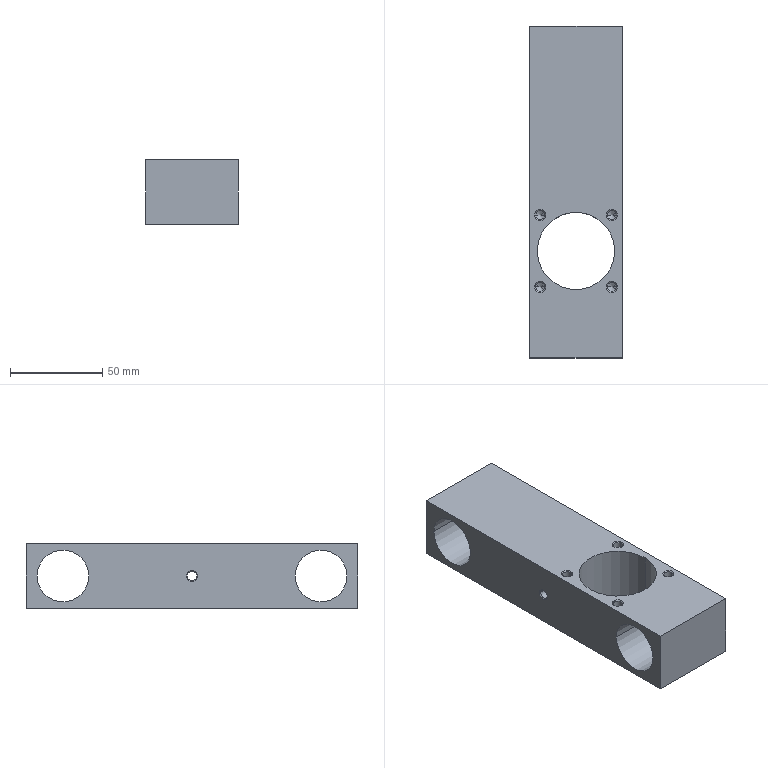Component | SolidWorks | DoubleFilmTransport-1_GuidePlate-1 | 1 solid | 40 faces | box 50 x 180 x 35 mm | volume 202252 mm3 | cone 18 | cylinder 16 | plane 6 | commonest cylinder face diameters 5 x10 28 x4 42 x2
STEP:
#1=COLOUR_RGB('',0.7922,0.8196,0.9333);
#2=FILL_AREA_STYLE_COLOUR('',#1);
#3=FILL_AREA_STYLE('',(#2));
#4=SURFACE_STYLE_FILL_AREA(#3);
#5=SURFACE_SIDE_STYLE('',(#4));
#6=SURFACE_STYLE_USAGE(.BOTH.,#5);
#7=PRESENTATION_STYLE_ASSIGNMENT((#6));
#8=CARTESIAN_POINT('',(-14.281,2.517,1.2));
#9=VERTEX_POINT('',#8);
#10=CARTESIAN_POINT('',(-14.478,2.517,1.2));
#11=VERTEX_POINT('',#10);
#12=CARTESIAN_POINT('',(-14.379,2.517,1.2));
#13=DIRECTION('',(0.,0.,1.));
#14=DIRECTION('',(-1.,0.,0.));
#15=AXIS2_PLACEMENT_3D('',#12,#13,#14);
#16=CIRCLE('',#15,0.09843);
#17=EDGE_CURVE('',#9,#11,#16,.T.);
#18=ORIENTED_EDGE('',*,*,#17,.F.);
#19=CARTESIAN_POINT('',(-14.26,2.517,1.22));
#20=VERTEX_POINT('',#19);
#21=CARTESIAN_POINT('',(-14.281,2.517,1.2));
#22=DIRECTION('',(0.7071,0.,0.7071));
#23=VECTOR('',#22,39.37);
#24=LINE('',#21,#23);
#25=EDGE_CURVE('',#9,#20,#24,.T.);
#26=ORIENTED_EDGE('',*,*,#25,.T.);
#27=CARTESIAN_POINT('',(-14.498,2.517,1.22));
#28=VERTEX_POINT('',#27);
#29=CARTESIAN_POINT('',(-14.379,2.517,1.22));
#30=DIRECTION('',(0.,0.,-1.));
#31=DIRECTION('',(-1.,0.,0.));
#32=AXIS2_PLACEMENT_3D('',#29,#30,#31);
#33=CIRCLE('',#32,0.1191);
#34=EDGE_CURVE('',#28,#20,#33,.T.);
#35=ORIENTED_EDGE('',*,*,#34,.F.);
#36=CARTESIAN_POINT('',(-14.478,2.517,1.2));
#37=DIRECTION('',(-0.7071,-0.,0.7071));
#38=VECTOR('',#37,39.37);
#39=LINE('',#36,#38);
#40=EDGE_CURVE('',#11,#28,#39,.T.);
#41=ORIENTED_EDGE('',*,*,#40,.F.);
#42=EDGE_LOOP('',(#18,#26,#35,#41));
#43=FACE_OUTER_BOUND('',#42,.T.);
#44=CARTESIAN_POINT('',(-14.379,2.517,1.2));
#45=DIRECTION('',(0.,0.,1.));
#46=DIRECTION('',(-1.,0.,0.));
#47=AXIS2_PLACEMENT_3D('',#44,#45,#46);
#48=CONICAL_SURFACE('',#47,0.09843,0.7854);
#49=ADVANCED_FACE('',(#43),#48,.F.);
#50=CARTESIAN_POINT('',(-15.812,2.517,1.2));
#51=VERTEX_POINT('',#50);
#52=CARTESIAN_POINT('',(-16.009,2.517,1.2));
#53=VERTEX_POINT('',#52);
#54=CARTESIAN_POINT('',(-15.91,2.517,1.2));
#55=DIRECTION('',(0.,0.,1.));
#56=DIRECTION('',(-1.,0.,0.));
#57=AXIS2_PLACEMENT_3D('',#54,#55,#56);
#58=CIRCLE('',#57,0.09843);
#59=EDGE_CURVE('',#51,#53,#58,.T.);
#60=ORIENTED_EDGE('',*,*,#59,.F.);
#61=CARTESIAN_POINT('',(-15.791,2.517,1.22));
#62=VERTEX_POINT('',#61);
#63=CARTESIAN_POINT('',(-15.812,2.517,1.2));
#64=DIRECTION('',(0.7071,0.,0.7071));
#65=VECTOR('',#64,39.37);
#66=LINE('',#63,#65);
#67=EDGE_CURVE('',#51,#62,#66,.T.);
#68=ORIENTED_EDGE('',*,*,#67,.T.);
#69=CARTESIAN_POINT('',(-16.029,2.517,1.22));
#70=VERTEX_POINT('',#69);
#71=CARTESIAN_POINT('',(-15.91,2.517,1.22));
#72=DIRECTION('',(0.,0.,-1.));
#73=DIRECTION('',(-1.,0.,0.));
#74=AXIS2_PLACEMENT_3D('',#71,#72,#73);
#75=CIRCLE('',#74,0.1191);
#76=EDGE_CURVE('',#70,#62,#75,.T.);
#77=ORIENTED_EDGE('',*,*,#76,.F.);
#78=CARTESIAN_POINT('',(-16.009,2.517,1.2));
#79=DIRECTION('',(-0.7071,-0.,0.7071));
#80=VECTOR('',#79,39.37);
#81=LINE('',#78,#80);
#82=EDGE_CURVE('',#53,#70,#81,.T.);
#83=ORIENTED_EDGE('',*,*,#82,.F.);
#84=EDGE_LOOP('',(#60,#68,#77,#83));
#85=FACE_OUTER_BOUND('',#84,.T.);
#86=CARTESIAN_POINT('',(-15.91,2.517,1.2));
#87=DIRECTION('',(0.,0.,1.));
#88=DIRECTION('',(-1.,0.,0.));
#89=AXIS2_PLACEMENT_3D('',#86,#87,#88);
#90=CONICAL_SURFACE('',#89,0.09843,0.7854);
#91=ADVANCED_FACE('',(#85),#90,.F.);
#92=CARTESIAN_POINT('',(-16.108,4.641,0.5315));
#93=VERTEX_POINT('',#92);
#94=CARTESIAN_POINT('',(-16.108,4.444,0.5315));
#95=VERTEX_POINT('',#94);
#96=CARTESIAN_POINT('',(-16.108,4.542,0.5315));
#97=DIRECTION('',(-1.,-0.,0.));
#98=DIRECTION('',(0.,-1.,0.));
#99=AXIS2_PLACEMENT_3D('',#96,#97,#98);
#100=CIRCLE('',#99,0.09843);
#101=EDGE_CURVE('',#93,#95,#100,.T.);
#102=ORIENTED_EDGE('',*,*,#101,.F.);
#103=CARTESIAN_POINT('',(-16.129,4.661,0.5315));
#104=VERTEX_POINT('',#103);
#105=CARTESIAN_POINT('',(-16.108,4.641,0.5315));
#106=DIRECTION('',(-0.7071,0.7071,0.));
#107=VECTOR('',#106,39.37);
#108=LINE('',#105,#107);
#109=EDGE_CURVE('',#93,#104,#108,.T.);
#110=ORIENTED_EDGE('',*,*,#109,.T.);
#111=CARTESIAN_POINT('',(-16.129,4.423,0.5315));
#112=VERTEX_POINT('',#111);
#113=CARTESIAN_POINT('',(-16.129,4.542,0.5315));
#114=DIRECTION('',(1.,0.,0.));
#115=DIRECTION('',(0.,-1.,0.));
#116=AXIS2_PLACEMENT_3D('',#113,#114,#115);
#117=CIRCLE('',#116,0.1191);
#118=EDGE_CURVE('',#112,#104,#117,.T.);
#119=ORIENTED_EDGE('',*,*,#118,.F.);
#120=CARTESIAN_POINT('',(-16.108,4.444,0.5315));
#121=DIRECTION('',(-0.7071,-0.7071,0.));
#122=VECTOR('',#121,39.37);
#123=LINE('',#120,#122);
#124=EDGE_CURVE('',#95,#112,#123,.T.);
#125=ORIENTED_EDGE('',*,*,#124,.F.);
#126=EDGE_LOOP('',(#102,#110,#119,#125));
#127=FACE_OUTER_BOUND('',#126,.T.);
#128=CARTESIAN_POINT('',(-16.108,4.542,0.5315));
#129=DIRECTION('',(-1.,-0.,0.));
#130=DIRECTION('',(0.,-1.,0.));
#131=AXIS2_PLACEMENT_3D('',#128,#129,#130);
#132=CONICAL_SURFACE('',#131,0.09843,0.7854);
#133=ADVANCED_FACE('',(#127),#132,.F.);
#134=CARTESIAN_POINT('',(-15.812,4.048,1.2));
#135=VERTEX_POINT('',#134);
#136=CARTESIAN_POINT('',(-16.009,4.048,1.2));
#137=VERTEX_POINT('',#136);
#138=CARTESIAN_POINT('',(-15.91,4.048,1.2));
#139=DIRECTION('',(0.,0.,1.));
#140=DIRECTION('',(-1.,0.,0.));
#141=AXIS2_PLACEMENT_3D('',#138,#139,#140);
#142=CIRCLE('',#141,0.09843);
#143=EDGE_CURVE('',#135,#137,#142,.T.);
#144=ORIENTED_EDGE('',*,*,#143,.F.);
#145=CARTESIAN_POINT('',(-15.791,4.048,1.22));
#146=VERTEX_POINT('',#145);
#147=CARTESIAN_POINT('',(-15.812,4.048,1.2));
#148=DIRECTION('',(0.7071,0.,0.7071));
#149=VECTOR('',#148,39.37);
#150=LINE('',#147,#149);
#151=EDGE_CURVE('',#135,#146,#150,.T.);
#152=ORIENTED_EDGE('',*,*,#151,.T.);
#153=CARTESIAN_POINT('',(-16.029,4.048,1.22));
#154=VERTEX_POINT('',#153);
#155=CARTESIAN_POINT('',(-15.91,4.048,1.22));
#156=DIRECTION('',(0.,0.,-1.));
#157=DIRECTION('',(-1.,0.,0.));
#158=AXIS2_PLACEMENT_3D('',#155,#156,#157);
#159=CIRCLE('',#158,0.1191);
#160=EDGE_CURVE('',#154,#146,#159,.T.);
#161=ORIENTED_EDGE('',*,*,#160,.F.);
#162=CARTESIAN_POINT('',(-16.009,4.048,1.2));
#163=DIRECTION('',(-0.7071,-0.,0.7071));
#164=VECTOR('',#163,39.37);
#165=LINE('',#162,#164);
#166=EDGE_CURVE('',#137,#154,#165,.T.);
#167=ORIENTED_EDGE('',*,*,#166,.F.);
#168=EDGE_LOOP('',(#144,#152,#161,#167));
#169=FACE_OUTER_BOUND('',#168,.T.);
#170=CARTESIAN_POINT('',(-15.91,4.048,1.2));
#171=DIRECTION('',(0.,0.,1.));
#172=DIRECTION('',(-1.,0.,0.));
#173=AXIS2_PLACEMENT_3D('',#170,#171,#172);
#174=CONICAL_SURFACE('',#173,0.09843,0.7854);
#175=ADVANCED_FACE('',(#169),#174,.F.);
#176=CARTESIAN_POINT('',(-14.281,4.048,1.2));
#177=VERTEX_POINT('',#176);
#178=CARTESIAN_POINT('',(-14.478,4.048,1.2));
#179=VERTEX_POINT('',#178);
#180=CARTESIAN_POINT('',(-14.379,4.048,1.2));
#181=DIRECTION('',(0.,0.,1.));
#182=DIRECTION('',(-1.,0.,0.));
#183=AXIS2_PLACEMENT_3D('',#180,#181,#182);
#184=CIRCLE('',#183,0.09843);
#185=EDGE_CURVE('',#177,#179,#184,.T.);
#186=ORIENTED_EDGE('',*,*,#185,.F.);
#187=CARTESIAN_POINT('',(-14.26,4.048,1.22));
#188=VERTEX_POINT('',#187);
#189=CARTESIAN_POINT('',(-14.281,4.048,1.2));
#190=DIRECTION('',(0.7071,0.,0.7071));
#191=VECTOR('',#190,39.37);
#192=LINE('',#189,#191);
#193=EDGE_CURVE('',#177,#188,#192,.T.);
#194=ORIENTED_EDGE('',*,*,#193,.T.);
#195=CARTESIAN_POINT('',(-14.498,4.048,1.22));
#196=VERTEX_POINT('',#195);
#197=CARTESIAN_POINT('',(-14.379,4.048,1.22));
#198=DIRECTION('',(0.,0.,-1.));
#199=DIRECTION('',(-1.,0.,0.));
#200=AXIS2_PLACEMENT_3D('',#197,#198,#199);
#201=CIRCLE('',#200,0.1191);
#202=EDGE_CURVE('',#196,#188,#201,.T.);
#203=ORIENTED_EDGE('',*,*,#202,.F.);
#204=CARTESIAN_POINT('',(-14.478,4.048,1.2));
#205=DIRECTION('',(-0.7071,-0.,0.7071));
#206=VECTOR('',#205,39.37);
#207=LINE('',#204,#206);
#208=EDGE_CURVE('',#179,#196,#207,.T.);
#209=ORIENTED_EDGE('',*,*,#208,.F.);
#210=EDGE_LOOP('',(#186,#194,#203,#209));
#211=FACE_OUTER_BOUND('',#210,.T.);
#212=CARTESIAN_POINT('',(-14.379,4.048,1.2));
#213=DIRECTION('',(0.,0.,1.));
#214=DIRECTION('',(-1.,0.,0.));
#215=AXIS2_PLACEMENT_3D('',#212,#213,#214);
#216=CONICAL_SURFACE('',#215,0.09843,0.7854);
#217=ADVANCED_FACE('',(#211),#216,.F.);
#218=CARTESIAN_POINT('',(-15.812,4.048,0.3937));
#219=VERTEX_POINT('',#218);
#220=CARTESIAN_POINT('',(-16.009,4.048,0.3937));
#221=VERTEX_POINT('',#220);
#222=CARTESIAN_POINT('',(-15.91,4.048,0.3937));
#223=DIRECTION('',(0.,0.,1.));
#224=DIRECTION('',(-1.,0.,0.));
#225=AXIS2_PLACEMENT_3D('',#222,#223,#224);
#226=CIRCLE('',#225,0.09843);
#227=EDGE_CURVE('',#219,#221,#226,.T.);
#228=ORIENTED_EDGE('',*,*,#227,.F.);
#229=CARTESIAN_POINT('',(-15.812,4.048,1.22));
#230=DIRECTION('',(0.,0.,1.));
#231=VECTOR('',#230,39.37);
#232=LINE('',#229,#231);
#233=EDGE_CURVE('',#219,#135,#232,.T.);
#234=ORIENTED_EDGE('',*,*,#233,.T.);
#235=ORIENTED_EDGE('',*,*,#143,.T.);
#236=CARTESIAN_POINT('',(-16.009,4.048,1.22));
#237=DIRECTION('',(0.,0.,1.));
#238=VECTOR('',#237,39.37);
#239=LINE('',#236,#238);
#240=EDGE_CURVE('',#221,#137,#239,.T.);
#241=ORIENTED_EDGE('',*,*,#240,.F.);
#242=EDGE_LOOP('',(#228,#234,#235,#241));
#243=FACE_OUTER_BOUND('',#242,.T.);
#244=CARTESIAN_POINT('',(-15.91,4.048,1.22));
#245=DIRECTION('',(0.,0.,1.));
#246=DIRECTION('',(-1.,0.,0.));
#247=AXIS2_PLACEMENT_3D('',#244,#245,#246);
#248=CYLINDRICAL_SURFACE('',#247,0.09843);
#249=ADVANCED_FACE('',(#243),#248,.F.);
#250=CARTESIAN_POINT('',(-15.91,4.048,0.3346));
#251=VERTEX_POINT('',#250);
#252=CARTESIAN_POINT('',(-16.009,4.048,0.3937));
#253=DIRECTION('',(-0.8572,-0.,0.515));
#254=VECTOR('',#253,39.37);
#255=LINE('',#252,#254);
#256=EDGE_CURVE('',#251,#221,#255,.T.);
#257=ORIENTED_EDGE('',*,*,#256,.F.);
#258=CARTESIAN_POINT('',(-15.812,4.048,0.3937));
#259=DIRECTION('',(0.8572,0.,0.515));
#260=VECTOR('',#259,39.37);
#261=LINE('',#258,#260);
#262=EDGE_CURVE('',#251,#219,#261,.T.);
#263=ORIENTED_EDGE('',*,*,#262,.T.);
#264=ORIENTED_EDGE('',*,*,#227,.T.);
#265=EDGE_LOOP('',(#257,#263,#264));
#266=FACE_OUTER_BOUND('',#265,.T.);
#267=CARTESIAN_POINT('',(-15.91,4.048,0.3937));
#268=DIRECTION('',(0.,0.,1.));
#269=DIRECTION('',(-1.,0.,0.));
#270=AXIS2_PLACEMENT_3D('',#267,#268,#269);
#271=CONICAL_SURFACE('',#270,0.09843,1.03);
#272=ADVANCED_FACE('',(#266),#271,.F.);
#273=CARTESIAN_POINT('',(-15.812,2.517,0.3937));
#274=VERTEX_POINT('',#273);
#275=CARTESIAN_POINT('',(-16.009,2.517,0.3937));
#276=VERTEX_POINT('',#275);
#277=CARTESIAN_POINT('',(-15.91,2.517,0.3937));
#278=DIRECTION('',(0.,0.,1.));
#279=DIRECTION('',(-1.,0.,0.));
#280=AXIS2_PLACEMENT_3D('',#277,#278,#279);
#281=CIRCLE('',#280,0.09843);
#282=EDGE_CURVE('',#274,#276,#281,.T.);
#283=ORIENTED_EDGE('',*,*,#282,.F.);
#284=CARTESIAN_POINT('',(-15.812,2.517,1.22));
#285=DIRECTION('',(0.,0.,1.));
#286=VECTOR('',#285,39.37);
#287=LINE('',#284,#286);
#288=EDGE_CURVE('',#274,#51,#287,.T.);
#289=ORIENTED_EDGE('',*,*,#288,.T.);
#290=ORIENTED_EDGE('',*,*,#59,.T.);
#291=CARTESIAN_POINT('',(-16.009,2.517,1.22));
#292=DIRECTION('',(0.,0.,1.));
#293=VECTOR('',#292,39.37);
#294=LINE('',#291,#293);
#295=EDGE_CURVE('',#276,#53,#294,.T.);
#296=ORIENTED_EDGE('',*,*,#295,.F.);
#297=EDGE_LOOP('',(#283,#289,#290,#296));
#298=FACE_OUTER_BOUND('',#297,.T.);
#299=CARTESIAN_POINT('',(-15.91,2.517,1.22));
#300=DIRECTION('',(0.,0.,1.));
#301=DIRECTION('',(-1.,0.,0.));
#302=AXIS2_PLACEMENT_3D('',#299,#300,#301);
#303=CYLINDRICAL_SURFACE('',#302,0.09843);
#304=ADVANCED_FACE('',(#298),#303,.F.);
#305=CARTESIAN_POINT('',(-15.91,2.517,0.3346));
#306=VERTEX_POINT('',#305);
#307=CARTESIAN_POINT('',(-16.009,2.517,0.3937));
#308=DIRECTION('',(-0.8572,-0.,0.515));
#309=VECTOR('',#308,39.37);
#310=LINE('',#307,#309);
#311=EDGE_CURVE('',#306,#276,#310,.T.);
#312=ORIENTED_EDGE('',*,*,#311,.F.);
#313=CARTESIAN_POINT('',(-15.812,2.517,0.3937));
#314=DIRECTION('',(0.8572,0.,0.515));
#315=VECTOR('',#314,39.37);
#316=LINE('',#313,#315);
#317=EDGE_CURVE('',#306,#274,#316,.T.);
#318=ORIENTED_EDGE('',*,*,#317,.T.);
#319=ORIENTED_EDGE('',*,*,#282,.T.);
#320=EDGE_LOOP('',(#312,#318,#319));
#321=FACE_OUTER_BOUND('',#320,.T.);
#322=CARTESIAN_POINT('',(-15.91,2.517,0.3937));
#323=DIRECTION('',(0.,0.,1.));
#324=DIRECTION('',(-1.,0.,0.));
#325=AXIS2_PLACEMENT_3D('',#322,#323,#324);
#326=CONICAL_SURFACE('',#325,0.09843,1.03);
#327=ADVANCED_FACE('',(#321),#326,.F.);
#328=CARTESIAN_POINT('',(-14.281,2.517,0.3937));
#329=VERTEX_POINT('',#328);
#330=CARTESIAN_POINT('',(-14.478,2.517,0.3937));
#331=VERTEX_POINT('',#330);
#332=CARTESIAN_POINT('',(-14.379,2.517,0.3937));
#333=DIRECTION('',(0.,0.,1.));
#334=DIRECTION('',(-1.,0.,0.));
#335=AXIS2_PLACEMENT_3D('',#332,#333,#334);
#336=CIRCLE('',#335,0.09843);
#337=EDGE_CURVE('',#329,#331,#336,.T.);
#338=ORIENTED_EDGE('',*,*,#337,.F.);
#339=CARTESIAN_POINT('',(-14.281,2.517,1.22));
#340=DIRECTION('',(0.,0.,1.));
#341=VECTOR('',#340,39.37);
#342=LINE('',#339,#341);
#343=EDGE_CURVE('',#329,#9,#342,.T.);
#344=ORIENTED_EDGE('',*,*,#343,.T.);
#345=ORIENTED_EDGE('',*,*,#17,.T.);
#346=CARTESIAN_POINT('',(-14.478,2.517,1.22));
#347=DIRECTION('',(0.,0.,1.));
#348=VECTOR('',#347,39.37);
#349=LINE('',#346,#348);
#350=EDGE_CURVE('',#331,#11,#349,.T.);
#351=ORIENTED_EDGE('',*,*,#350,.F.);
#352=EDGE_LOOP('',(#338,#344,#345,#351));
#353=FACE_OUTER_BOUND('',#352,.T.);
#354=CARTESIAN_POINT('',(-14.379,2.517,1.22));
#355=DIRECTION('',(0.,0.,1.));
#356=DIRECTION('',(-1.,0.,0.));
#357=AXIS2_PLACEMENT_3D('',#354,#355,#356);
#358=CYLINDRICAL_SURFACE('',#357,0.09843);
#359=ADVANCED_FACE('',(#353),#358,.F.);
#360=CARTESIAN_POINT('',(-14.379,2.517,0.3346));
#361=VERTEX_POINT('',#360);
#362=CARTESIAN_POINT('',(-14.478,2.517,0.3937));
#363=DIRECTION('',(-0.8572,-0.,0.515));
#364=VECTOR('',#363,39.37);
#365=LINE('',#362,#364);
#366=EDGE_CURVE('',#361,#331,#365,.T.);
#367=ORIENTED_EDGE('',*,*,#366,.F.);
#368=CARTESIAN_POINT('',(-14.281,2.517,0.3937));
#369=DIRECTION('',(0.8572,0.,0.515));
#370=VECTOR('',#369,39.37);
#371=LINE('',#368,#370);
#372=EDGE_CURVE('',#361,#329,#371,.T.);
#373=ORIENTED_EDGE('',*,*,#372,.T.);
#374=ORIENTED_EDGE('',*,*,#337,.T.);
#375=EDGE_LOOP('',(#367,#373,#374));
#376=FACE_OUTER_BOUND('',#375,.T.);
#377=CARTESIAN_POINT('',(-14.379,2.517,0.3937));
#378=DIRECTION('',(0.,0.,1.));
#379=DIRECTION('',(-1.,0.,0.));
#380=AXIS2_PLACEMENT_3D('',#377,#378,#379);
#381=CONICAL_SURFACE('',#380,0.09843,1.03);
#382=ADVANCED_FACE('',(#376),#381,.F.);
#383=CARTESIAN_POINT('',(-14.281,4.048,0.3937));
#384=VERTEX_POINT('',#383);
#385=CARTESIAN_POINT('',(-14.478,4.048,0.3937));
#386=VERTEX_POINT('',#385);
#387=CARTESIAN_POINT('',(-14.379,4.048,0.3937));
#388=DIRECTION('',(0.,0.,1.));
#389=DIRECTION('',(-1.,0.,0.));
#390=AXIS2_PLACEMENT_3D('',#387,#388,#389);
#391=CIRCLE('',#390,0.09843);
#392=EDGE_CURVE('',#384,#386,#391,.T.);
#393=ORIENTED_EDGE('',*,*,#392,.F.);
#394=CARTESIAN_POINT('',(-14.281,4.048,1.22));
#395=DIRECTION('',(0.,0.,1.));
#396=VECTOR('',#395,39.37);
#397=LINE('',#394,#396);
#398=EDGE_CURVE('',#384,#177,#397,.T.);
#399=ORIENTED_EDGE('',*,*,#398,.T.);
#400=ORIENTED_EDGE('',*,*,#185,.T.);
#401=CARTESIAN_POINT('',(-14.478,4.048,1.22));
#402=DIRECTION('',(0.,0.,1.));
#403=VECTOR('',#402,39.37);
#404=LINE('',#401,#403);
#405=EDGE_CURVE('',#386,#179,#404,.T.);
#406=ORIENTED_EDGE('',*,*,#405,.F.);
#407=EDGE_LOOP('',(#393,#399,#400,#406));
#408=FACE_OUTER_BOUND('',#407,.T.);
#409=CARTESIAN_POINT('',(-14.379,4.048,1.22));
#410=DIRECTION('',(0.,0.,1.));
#411=DIRECTION('',(-1.,0.,0.));
#412=AXIS2_PLACEMENT_3D('',#409,#410,#411);
#413=CYLINDRICAL_SURFACE('',#412,0.09843);
#414=ADVANCED_FACE('',(#408),#413,.F.);
#415=CARTESIAN_POINT('',(-14.379,4.048,0.3346));
#416=VERTEX_POINT('',#415);
#417=CARTESIAN_POINT('',(-14.478,4.048,0.3937));
#418=DIRECTION('',(-0.8572,-0.,0.515));
#419=VECTOR('',#418,39.37);
#420=LINE('',#417,#419);
#421=EDGE_CURVE('',#416,#386,#420,.T.);
#422=ORIENTED_EDGE('',*,*,#421,.F.);
#423=CARTESIAN_POINT('',(-14.281,4.048,0.3937));
#424=DIRECTION('',(0.8572,0.,0.515));
#425=VECTOR('',#424,39.37);
#426=LINE('',#423,#425);
#427=EDGE_CURVE('',#416,#384,#426,.T.);
#428=ORIENTED_EDGE('',*,*,#427,.T.);
#429=ORIENTED_EDGE('',*,*,#392,.T.);
#430=EDGE_LOOP('',(#422,#428,#429));
#431=FACE_OUTER_BOUND('',#430,.T.);
#432=CARTESIAN_POINT('',(-14.379,4.048,0.3937));
#433=DIRECTION('',(0.,0.,1.));
#434=DIRECTION('',(-1.,0.,0.));
#435=AXIS2_PLACEMENT_3D('',#432,#433,#434);
#436=CONICAL_SURFACE('',#435,0.09843,1.03);
#437=ADVANCED_FACE('',(#431),#436,.F.);
#438=CARTESIAN_POINT('',(-14.161,4.641,0.5315));
#439=VERTEX_POINT('',#438);
#440=CARTESIAN_POINT('',(-14.161,4.444,0.5315));
#441=VERTEX_POINT('',#440);
#442=CARTESIAN_POINT('',(-14.161,4.542,0.5315));
#443=DIRECTION('',(-1.,-0.,0.));
#444=DIRECTION('',(0.,-1.,0.));
#445=AXIS2_PLACEMENT_3D('',#442,#443,#444);
#446=CIRCLE('',#445,0.09843);
#447=EDGE_CURVE('',#439,#441,#446,.T.);
#448=ORIENTED_EDGE('',*,*,#447,.F.);
#449=CARTESIAN_POINT('',(-16.129,4.641,0.5315));
#450=DIRECTION('',(-1.,-0.,0.));
#451=VECTOR('',#450,39.37);
#452=LINE('',#449,#451);
#453=EDGE_CURVE('',#439,#93,#452,.T.);
#454=ORIENTED_EDGE('',*,*,#453,.T.);
#455=ORIENTED_EDGE('',*,*,#101,.T.);
#456=CARTESIAN_POINT('',(-16.129,4.444,0.5315));
#457=DIRECTION('',(-1.,-0.,0.));
#458=VECTOR('',#457,39.37);
#459=LINE('',#456,#458);
#460=EDGE_CURVE('',#441,#95,#459,.T.);
#461=ORIENTED_EDGE('',*,*,#460,.F.);
#462=EDGE_LOOP('',(#448,#454,#455,#461));
#463=FACE_OUTER_BOUND('',#462,.T.);
#464=CARTESIAN_POINT('',(-16.129,4.542,0.5315));
#465=DIRECTION('',(-1.,-0.,0.));
#466=DIRECTION('',(0.,-1.,0.));
#467=AXIS2_PLACEMENT_3D('',#464,#465,#466);
#468=CYLINDRICAL_SURFACE('',#467,0.09843);
#469=ADVANCED_FACE('',(#463),#468,.F.);
#470=CARTESIAN_POINT('',(-14.161,2.338,0.5315));
#471=VERTEX_POINT('',#470);
#472=CARTESIAN_POINT('',(-14.161,1.235,0.5315));
#473=VERTEX_POINT('',#472);
#474=CARTESIAN_POINT('',(-14.161,1.786,0.5315));
#475=DIRECTION('',(-1.,-0.,0.));
#476=DIRECTION('',(0.,-1.,0.));
#477=AXIS2_PLACEMENT_3D('',#474,#475,#476);
#478=CIRCLE('',#477,0.5512);
#479=EDGE_CURVE('',#471,#473,#478,.T.);
#480=ORIENTED_EDGE('',*,*,#479,.F.);
#481=CARTESIAN_POINT('',(-16.129,2.338,0.5315));
#482=VERTEX_POINT('',#481);
#483=CARTESIAN_POINT('',(-16.129,2.338,0.5315));
#484=DIRECTION('',(-1.,-0.,0.));
#485=VECTOR('',#484,39.37);
#486=LINE('',#483,#485);
#487=EDGE_CURVE('',#471,#482,#486,.T.);
#488=ORIENTED_EDGE('',*,*,#487,.T.);
#489=CARTESIAN_POINT('',(-16.129,1.235,0.5315));
#490=VERTEX_POINT('',#489);
#491=CARTESIAN_POINT('',(-16.129,1.786,0.5315));
#492=DIRECTION('',(-1.,-0.,0.));
#493=DIRECTION('',(0.,-1.,0.));
#494=AXIS2_PLACEMENT_3D('',#491,#492,#493);
#495=CIRCLE('',#494,0.5512);
#496=EDGE_CURVE('',#482,#490,#495,.T.);
#497=ORIENTED_EDGE('',*,*,#496,.T.);
#498=CARTESIAN_POINT('',(-16.129,1.235,0.5315));
#499=DIRECTION('',(-1.,-0.,0.));
#500=VECTOR('',#499,39.37);
#501=LINE('',#498,#500);
#502=EDGE_CURVE('',#473,#490,#501,.T.);
#503=ORIENTED_EDGE('',*,*,#502,.F.);
#504=EDGE_LOOP('',(#480,#488,#497,#503));
#505=FACE_OUTER_BOUND('',#504,.T.);
#506=CARTESIAN_POINT('',(-16.129,1.786,0.5315));
#507=DIRECTION('',(-1.,-0.,0.));
#508=DIRECTION('',(0.,-1.,0.));
#509=AXIS2_PLACEMENT_3D('',#506,#507,#508);
#510=CYLINDRICAL_SURFACE('',#509,0.5512);
#511=ADVANCED_FACE('',(#505),#510,.F.);
#512=CARTESIAN_POINT('',(-14.161,7.849,0.5315));
#513=VERTEX_POINT('',#512);
#514=CARTESIAN_POINT('',(-14.161,6.747,0.5315));
#515=VERTEX_POINT('',#514);
#516=CARTESIAN_POINT('',(-14.161,7.298,0.5315));
#517=DIRECTION('',(-1.,-0.,0.));
#518=DIRECTION('',(0.,-1.,0.));
#519=AXIS2_PLACEMENT_3D('',#516,#517,#518);
#520=CIRCLE('',#519,0.5512);
#521=EDGE_CURVE('',#513,#515,#520,.T.);
#522=ORIENTED_EDGE('',*,*,#521,.F.);
#523=CARTESIAN_POINT('',(-16.129,7.849,0.5315));
#524=VERTEX_POINT('',#523);
#525=CARTESIAN_POINT('',(-16.129,7.849,0.5315));
#526=DIRECTION('',(-1.,-0.,0.));
#527=VECTOR('',#526,39.37);
#528=LINE('',#525,#527);
#529=EDGE_CURVE('',#513,#524,#528,.T.);
#530=ORIENTED_EDGE('',*,*,#529,.T.);
#531=CARTESIAN_POINT('',(-16.129,6.747,0.5315));
#532=VERTEX_POINT('',#531);
#533=CARTESIAN_POINT('',(-16.129,7.298,0.5315));
#534=DIRECTION('',(-1.,-0.,0.));
#535=DIRECTION('',(0.,-1.,0.));
#536=AXIS2_PLACEMENT_3D('',#533,#534,#535);
#537=CIRCLE('',#536,0.5512);
#538=EDGE_CURVE('',#524,#532,#537,.T.);
#539=ORIENTED_EDGE('',*,*,#538,.T.);
#540=CARTESIAN_POINT('',(-16.129,6.747,0.5315));
#541=DIRECTION('',(-1.,-0.,0.));
#542=VECTOR('',#541,39.37);
#543=LINE('',#540,#542);
#544=EDGE_CURVE('',#515,#532,#543,.T.);
#545=ORIENTED_EDGE('',*,*,#544,.F.);
#546=EDGE_LOOP('',(#522,#530,#539,#545));
#547=FACE_OUTER_BOUND('',#546,.T.);
#548=CARTESIAN_POINT('',(-16.129,7.298,0.5315));
#549=DIRECTION('',(-1.,-0.,0.));
#550=DIRECTION('',(0.,-1.,0.));
#551=AXIS2_PLACEMENT_3D('',#548,#549,#550);
#552=CYLINDRICAL_SURFACE('',#551,0.5512);
#553=ADVANCED_FACE('',(#547),#552,.F.);
#554=CARTESIAN_POINT('',(-15.972,3.282,1.22));
#555=VERTEX_POINT('',#554);
#556=CARTESIAN_POINT('',(-14.318,3.282,1.22));
#557=VERTEX_POINT('',#556);
#558=CARTESIAN_POINT('',(-15.145,3.282,1.22));
#559=DIRECTION('',(0.,0.,-1.));
#560=DIRECTION('',(1.,0.,0.));
#561=AXIS2_PLACEMENT_3D('',#558,#559,#560);
#562=CIRCLE('',#561,0.8268);
#563=EDGE_CURVE('',#555,#557,#562,.T.);
#564=ORIENTED_EDGE('',*,*,#563,.F.);
#565=CARTESIAN_POINT('',(-15.972,3.282,-0.1575));
#566=VERTEX_POINT('',#565);
#567=CARTESIAN_POINT('',(-15.972,3.282,-0.1575));
#568=DIRECTION('',(0.,0.,-1.));
#569=VECTOR('',#568,39.37);
#570=LINE('',#567,#569);
#571=EDGE_CURVE('',#555,#566,#570,.T.);
#572=ORIENTED_EDGE('',*,*,#571,.T.);
#573=CARTESIAN_POINT('',(-14.318,3.282,-0.1575));
#574=VERTEX_POINT('',#573);
#575=CARTESIAN_POINT('',(-15.145,3.282,-0.1575));
#576=DIRECTION('',(0.,0.,-1.));
#577=DIRECTION('',(1.,0.,0.));
#578=AXIS2_PLACEMENT_3D('',#575,#576,#577);
#579=CIRCLE('',#578,0.8268);
#580=EDGE_CURVE('',#566,#574,#579,.T.);
#581=ORIENTED_EDGE('',*,*,#580,.T.);
#582=CARTESIAN_POINT('',(-14.318,3.282,-0.1575));
#583=DIRECTION('',(0.,0.,-1.));
#584=VECTOR('',#583,39.37);
#585=LINE('',#582,#584);
#586=EDGE_CURVE('',#557,#574,#585,.T.);
#587=ORIENTED_EDGE('',*,*,#586,.F.);
#588=EDGE_LOOP('',(#564,#572,#581,#587));
#589=FACE_OUTER_BOUND('',#588,.T.);
#590=CARTESIAN_POINT('',(-15.145,3.282,-0.1575));
#591=DIRECTION('',(0.,0.,-1.));
#592=DIRECTION('',(1.,0.,0.));
#593=AXIS2_PLACEMENT_3D('',#590,#591,#592);
#594=CYLINDRICAL_SURFACE('',#593,0.8268);
#595=ADVANCED_FACE('',(#589),#594,.F.);
#596=CARTESIAN_POINT('',(-14.161,8.086,1.22));
#597=VERTEX_POINT('',#596);
#598=CARTESIAN_POINT('',(-16.129,8.086,1.22));
#599=VERTEX_POINT('',#598);
#600=CARTESIAN_POINT('',(-14.161,8.086,1.22));
#601=DIRECTION('',(-1.,-0.,0.));
#602=VECTOR('',#601,39.37);
#603=LINE('',#600,#602);
#604=EDGE_CURVE('',#597,#599,#603,.T.);
#605=ORIENTED_EDGE('',*,*,#604,.F.);
#606=CARTESIAN_POINT('',(-14.161,8.086,-0.1575));
#607=VERTEX_POINT('',#606);
#608=CARTESIAN_POINT('',(-14.161,8.086,-0.1575));
#609=DIRECTION('',(0.,0.,1.));
#610=VECTOR('',#609,39.37);
#611=LINE('',#608,#610);
#612=EDGE_CURVE('',#607,#597,#611,.T.);
#613=ORIENTED_EDGE('',*,*,#612,.F.);
#614=CARTESIAN_POINT('',(-16.129,8.086,-0.1575));
#615=VERTEX_POINT('',#614);
#616=CARTESIAN_POINT('',(-14.161,8.086,-0.1575));
#617=DIRECTION('',(-1.,-0.,0.));
#618=VECTOR('',#617,39.37);
#619=LINE('',#616,#618);
#620=EDGE_CURVE('',#607,#615,#619,.T.);
#621=ORIENTED_EDGE('',*,*,#620,.T.);
#622=CARTESIAN_POINT('',(-16.129,8.086,-0.1575));
#623=DIRECTION('',(0.,0.,1.));
#624=VECTOR('',#623,39.37);
#625=LINE('',#622,#624);
#626=EDGE_CURVE('',#615,#599,#625,.T.);
#627=ORIENTED_EDGE('',*,*,#626,.T.);
#628=EDGE_LOOP('',(#605,#613,#621,#627));
#629=FACE_OUTER_BOUND('',#628,.T.);
#630=CARTESIAN_POINT('',(-14.161,8.086,-0.1575));
#631=DIRECTION('',(-0.,1.,0.));
#632=DIRECTION('',(-1.,-0.,0.));
#633=AXIS2_PLACEMENT_3D('',#630,#631,#632);
#634=PLANE('',#633);
#635=ADVANCED_FACE('',(#629),#634,.T.);
#636=CARTESIAN_POINT('',(-14.161,4.542,0.5315));
#637=DIRECTION('',(-1.,-0.,0.));
#638=DIRECTION('',(0.,-1.,0.));
#639=AXIS2_PLACEMENT_3D('',#636,#637,#638);
#640=CIRCLE('',#639,0.09843);
#641=EDGE_CURVE('',#441,#439,#640,.T.);
#642=ORIENTED_EDGE('',*,*,#641,.T.);
#643=ORIENTED_EDGE('',*,*,#447,.T.);
#644=EDGE_LOOP('',(#642,#643));
#645=FACE_BOUND('',#644,.T.);
#646=CARTESIAN_POINT('',(-14.161,1.786,0.5315));
#647=DIRECTION('',(-1.,-0.,0.));
#648=DIRECTION('',(0.,-1.,0.));
#649=AXIS2_PLACEMENT_3D('',#646,#647,#648);
#650=CIRCLE('',#649,0.5512);
#651=EDGE_CURVE('',#473,#471,#650,.T.);
#652=ORIENTED_EDGE('',*,*,#651,.T.);
#653=ORIENTED_EDGE('',*,*,#479,.T.);
#654=EDGE_LOOP('',(#652,#653));
#655=FACE_BOUND('',#654,.T.);
#656=CARTESIAN_POINT('',(-14.161,7.298,0.5315));
#657=DIRECTION('',(-1.,-0.,0.));
#658=DIRECTION('',(0.,-1.,0.));
#659=AXIS2_PLACEMENT_3D('',#656,#657,#658);
#660=CIRCLE('',#659,0.5512);
#661=EDGE_CURVE('',#515,#513,#660,.T.);
#662=ORIENTED_EDGE('',*,*,#661,.T.);
#663=ORIENTED_EDGE('',*,*,#521,.T.);
#664=EDGE_LOOP('',(#662,#663));
#665=FACE_BOUND('',#664,.T.);
#666=CARTESIAN_POINT('',(-14.161,0.999,1.22));
#667=VERTEX_POINT('',#666);
#668=CARTESIAN_POINT('',(-14.161,0.999,1.22));
#669=DIRECTION('',(-0.,1.,0.));
#670=VECTOR('',#669,39.37);
#671=LINE('',#668,#670);
#672=EDGE_CURVE('',#667,#597,#671,.T.);
#673=ORIENTED_EDGE('',*,*,#672,.F.);
#674=CARTESIAN_POINT('',(-14.161,0.999,-0.1575));
#675=VERTEX_POINT('',#674);
#676=CARTESIAN_POINT('',(-14.161,0.999,-0.1575));
#677=DIRECTION('',(0.,0.,1.));
#678=VECTOR('',#677,39.37);
#679=LINE('',#676,#678);
#680=EDGE_CURVE('',#675,#667,#679,.T.);
#681=ORIENTED_EDGE('',*,*,#680,.F.);
#682=CARTESIAN_POINT('',(-14.161,0.999,-0.1575));
#683=DIRECTION('',(-0.,1.,0.));
#684=VECTOR('',#683,39.37);
#685=LINE('',#682,#684);
#686=EDGE_CURVE('',#675,#607,#685,.T.);
#687=ORIENTED_EDGE('',*,*,#686,.T.);
#688=ORIENTED_EDGE('',*,*,#612,.T.);
#689=EDGE_LOOP('',(#673,#681,#687,#688));
#690=FACE_OUTER_BOUND('',#689,.T.);
#691=CARTESIAN_POINT('',(-14.161,0.999,-0.1575));
#692=DIRECTION('',(1.,0.,0.));
#693=DIRECTION('',(-0.,1.,0.));
#694=AXIS2_PLACEMENT_3D('',#691,#692,#693);
#695=PLANE('',#694);
#696=ADVANCED_FACE('',(#645,#655,#665,#690),#695,.T.);
#697=CARTESIAN_POINT('',(-16.129,0.999,1.22));
#698=VERTEX_POINT('',#697);
#699=CARTESIAN_POINT('',(-16.129,0.999,1.22));
#700=DIRECTION('',(1.,0.,0.));
#701=VECTOR('',#700,39.37);
#702=LINE('',#699,#701);
#703=EDGE_CURVE('',#698,#667,#702,.T.);
#704=ORIENTED_EDGE('',*,*,#703,.F.);
#705=CARTESIAN_POINT('',(-16.129,0.999,-0.1575));
#706=VERTEX_POINT('',#705);
#707=CARTESIAN_POINT('',(-16.129,0.999,-0.1575));
#708=DIRECTION('',(0.,0.,1.));
#709=VECTOR('',#708,39.37);
#710=LINE('',#707,#709);
#711=EDGE_CURVE('',#706,#698,#710,.T.);
#712=ORIENTED_EDGE('',*,*,#711,.F.);
#713=CARTESIAN_POINT('',(-16.129,0.999,-0.1575));
#714=DIRECTION('',(1.,0.,0.));
#715=VECTOR('',#714,39.37);
#716=LINE('',#713,#715);
#717=EDGE_CURVE('',#706,#675,#716,.T.);
#718=ORIENTED_EDGE('',*,*,#717,.T.);
#719=ORIENTED_EDGE('',*,*,#680,.T.);
#720=EDGE_LOOP('',(#704,#712,#718,#719));
#721=FACE_OUTER_BOUND('',#720,.T.);
#722=CARTESIAN_POINT('',(-16.129,0.999,-0.1575));
#723=DIRECTION('',(0.,-1.,0.));
#724=DIRECTION('',(1.,0.,0.));
#725=AXIS2_PLACEMENT_3D('',#722,#723,#724);
#726=PLANE('',#725);
#727=ADVANCED_FACE('',(#721),#726,.T.);
#728=ORIENTED_EDGE('',*,*,#118,.T.);
#729=CARTESIAN_POINT('',(-16.129,4.542,0.5315));
#730=DIRECTION('',(1.,0.,0.));
#731=DIRECTION('',(0.,-1.,0.));
#732=AXIS2_PLACEMENT_3D('',#729,#730,#731);
#733=CIRCLE('',#732,0.1191);
#734=EDGE_CURVE('',#104,#112,#733,.T.);
#735=ORIENTED_EDGE('',*,*,#734,.T.);
#736=EDGE_LOOP('',(#728,#735));
#737=FACE_BOUND('',#736,.T.);
#738=CARTESIAN_POINT('',(-16.129,1.786,0.5315));
#739=DIRECTION('',(-1.,-0.,0.));
#740=DIRECTION('',(0.,-1.,0.));
#741=AXIS2_PLACEMENT_3D('',#738,#739,#740);
#742=CIRCLE('',#741,0.5512);
#743=EDGE_CURVE('',#490,#482,#742,.T.);
#744=ORIENTED_EDGE('',*,*,#743,.F.);
#745=ORIENTED_EDGE('',*,*,#496,.F.);
#746=EDGE_LOOP('',(#744,#745));
#747=FACE_BOUND('',#746,.T.);
#748=CARTESIAN_POINT('',(-16.129,7.298,0.5315));
#749=DIRECTION('',(-1.,-0.,0.));
#750=DIRECTION('',(0.,-1.,0.));
#751=AXIS2_PLACEMENT_3D('',#748,#749,#750);
#752=CIRCLE('',#751,0.5512);
#753=EDGE_CURVE('',#532,#524,#752,.T.);
#754=ORIENTED_EDGE('',*,*,#753,.F.);
#755=ORIENTED_EDGE('',*,*,#538,.F.);
#756=EDGE_LOOP('',(#754,#755));
#757=FACE_BOUND('',#756,.T.);
#758=CARTESIAN_POINT('',(-16.129,8.086,1.22));
#759=DIRECTION('',(0.,-1.,0.));
#760=VECTOR('',#759,39.37);
#761=LINE('',#758,#760);
#762=EDGE_CURVE('',#599,#698,#761,.T.);
#763=ORIENTED_EDGE('',*,*,#762,.F.);
#764=ORIENTED_EDGE('',*,*,#626,.F.);
#765=CARTESIAN_POINT('',(-16.129,8.086,-0.1575));
#766=DIRECTION('',(0.,-1.,0.));
#767=VECTOR('',#766,39.37);
#768=LINE('',#765,#767);
#769=EDGE_CURVE('',#615,#706,#768,.T.);
#770=ORIENTED_EDGE('',*,*,#769,.T.);
#771=ORIENTED_EDGE('',*,*,#711,.T.);
#772=EDGE_LOOP('',(#763,#764,#770,#771));
#773=FACE_OUTER_BOUND('',#772,.T.);
#774=CARTESIAN_POINT('',(-16.129,8.086,-0.1575));
#775=DIRECTION('',(-1.,-0.,0.));
#776=DIRECTION('',(0.,-1.,0.));
#777=AXIS2_PLACEMENT_3D('',#774,#775,#776);
#778=PLANE('',#777);
#779=ADVANCED_FACE('',(#737,#747,#757,#773),#778,.T.);
#780=CARTESIAN_POINT('',(-15.145,3.282,-0.1575));
#781=DIRECTION('',(0.,0.,-1.));
#782=DIRECTION('',(1.,0.,0.));
#783=AXIS2_PLACEMENT_3D('',#780,#781,#782);
#784=CIRCLE('',#783,0.8268);
#785=EDGE_CURVE('',#574,#566,#784,.T.);
#786=ORIENTED_EDGE('',*,*,#785,.F.);
#787=ORIENTED_EDGE('',*,*,#580,.F.);
#788=EDGE_LOOP('',(#786,#787));
#789=FACE_BOUND('',#788,.T.);
#790=ORIENTED_EDGE('',*,*,#620,.F.);
#791=ORIENTED_EDGE('',*,*,#686,.F.);
#792=ORIENTED_EDGE('',*,*,#717,.F.);
#793=ORIENTED_EDGE('',*,*,#769,.F.);
#794=EDGE_LOOP('',(#790,#791,#792,#793));
#795=FACE_OUTER_BOUND('',#794,.T.);
#796=CARTESIAN_POINT('',(-15.145,4.542,-0.1575));
#797=DIRECTION('',(0.,0.,1.));
#798=DIRECTION('',(-1.,-0.,0.));
#799=AXIS2_PLACEMENT_3D('',#796,#797,#798);
#800=PLANE('',#799);
#801=ADVANCED_FACE('',(#789,#795),#800,.F.);
#802=ORIENTED_EDGE('',*,*,#202,.T.);
#803=CARTESIAN_POINT('',(-14.379,4.048,1.22));
#804=DIRECTION('',(0.,0.,-1.));
#805=DIRECTION('',(-1.,0.,0.));
#806=AXIS2_PLACEMENT_3D('',#803,#804,#805);
#807=CIRCLE('',#806,0.1191);
#808=EDGE_CURVE('',#188,#196,#807,.T.);
#809=ORIENTED_EDGE('',*,*,#808,.T.);
#810=EDGE_LOOP('',(#802,#809));
#811=FACE_BOUND('',#810,.T.);
#812=ORIENTED_EDGE('',*,*,#160,.T.);
#813=CARTESIAN_POINT('',(-15.91,4.048,1.22));
#814=DIRECTION('',(0.,0.,-1.));
#815=DIRECTION('',(-1.,0.,0.));
#816=AXIS2_PLACEMENT_3D('',#813,#814,#815);
#817=CIRCLE('',#816,0.1191);
#818=EDGE_CURVE('',#146,#154,#817,.T.);
#819=ORIENTED_EDGE('',*,*,#818,.T.);
#820=EDGE_LOOP('',(#812,#819));
#821=FACE_BOUND('',#820,.T.);
#822=ORIENTED_EDGE('',*,*,#76,.T.);
#823=CARTESIAN_POINT('',(-15.91,2.517,1.22));
#824=DIRECTION('',(0.,0.,-1.));
#825=DIRECTION('',(-1.,0.,0.));
#826=AXIS2_PLACEMENT_3D('',#823,#824,#825);
#827=CIRCLE('',#826,0.1191);
#828=EDGE_CURVE('',#62,#70,#827,.T.);
#829=ORIENTED_EDGE('',*,*,#828,.T.);
#830=EDGE_LOOP('',(#822,#829));
#831=FACE_BOUND('',#830,.T.);
#832=ORIENTED_EDGE('',*,*,#34,.T.);
#833=CARTESIAN_POINT('',(-14.379,2.517,1.22));
#834=DIRECTION('',(0.,0.,-1.));
#835=DIRECTION('',(-1.,0.,0.));
#836=AXIS2_PLACEMENT_3D('',#833,#834,#835);
#837=CIRCLE('',#836,0.1191);
#838=EDGE_CURVE('',#20,#28,#837,.T.);
#839=ORIENTED_EDGE('',*,*,#838,.T.);
#840=EDGE_LOOP('',(#832,#839));
#841=FACE_BOUND('',#840,.T.);
#842=CARTESIAN_POINT('',(-15.145,3.282,1.22));
#843=DIRECTION('',(0.,0.,-1.));
#844=DIRECTION('',(1.,0.,0.));
#845=AXIS2_PLACEMENT_3D('',#842,#843,#844);
#846=CIRCLE('',#845,0.8268);
#847=EDGE_CURVE('',#557,#555,#846,.T.);
#848=ORIENTED_EDGE('',*,*,#847,.T.);
#849=ORIENTED_EDGE('',*,*,#563,.T.);
#850=EDGE_LOOP('',(#848,#849));
#851=FACE_BOUND('',#850,.T.);
#852=ORIENTED_EDGE('',*,*,#604,.T.);
#853=ORIENTED_EDGE('',*,*,#762,.T.);
#854=ORIENTED_EDGE('',*,*,#703,.T.);
#855=ORIENTED_EDGE('',*,*,#672,.T.);
#856=EDGE_LOOP('',(#852,#853,#854,#855));
#857=FACE_OUTER_BOUND('',#856,.T.);
#858=CARTESIAN_POINT('',(-15.145,4.542,1.22));
#859=DIRECTION('',(0.,0.,1.));
#860=DIRECTION('',(-1.,-0.,0.));
#861=AXIS2_PLACEMENT_3D('',#858,#859,#860);
#862=PLANE('',#861);
#863=ADVANCED_FACE('',(#811,#821,#831,#841,#851,#857),#862,.T.);
#864=ORIENTED_EDGE('',*,*,#571,.F.);
#865=ORIENTED_EDGE('',*,*,#847,.F.);
#866=ORIENTED_EDGE('',*,*,#586,.T.);
#867=ORIENTED_EDGE('',*,*,#785,.T.);
#868=EDGE_LOOP('',(#864,#865,#866,#867));
#869=FACE_OUTER_BOUND('',#868,.T.);
#870=CARTESIAN_POINT('',(-15.145,3.282,-0.1575));
#871=DIRECTION('',(0.,0.,-1.));
#872=DIRECTION('',(1.,0.,0.));
#873=AXIS2_PLACEMENT_3D('',#870,#871,#872);
#874=CYLINDRICAL_SURFACE('',#873,0.8268);
#875=ADVANCED_FACE('',(#869),#874,.F.);
#876=ORIENTED_EDGE('',*,*,#529,.F.);
#877=ORIENTED_EDGE('',*,*,#661,.F.);
#878=ORIENTED_EDGE('',*,*,#544,.T.);
#879=ORIENTED_EDGE('',*,*,#753,.T.);
#880=EDGE_LOOP('',(#876,#877,#878,#879));
#881=FACE_OUTER_BOUND('',#880,.T.);
#882=CARTESIAN_POINT('',(-16.129,7.298,0.5315));
#883=DIRECTION('',(-1.,-0.,0.));
#884=DIRECTION('',(0.,-1.,0.));
#885=AXIS2_PLACEMENT_3D('',#882,#883,#884);
#886=CYLINDRICAL_SURFACE('',#885,0.5512);
#887=ADVANCED_FACE('',(#881),#886,.F.);
#888=ORIENTED_EDGE('',*,*,#487,.F.);
#889=ORIENTED_EDGE('',*,*,#651,.F.);
#890=ORIENTED_EDGE('',*,*,#502,.T.);
#891=ORIENTED_EDGE('',*,*,#743,.T.);
#892=EDGE_LOOP('',(#888,#889,#890,#891));
#893=FACE_OUTER_BOUND('',#892,.T.);
#894=CARTESIAN_POINT('',(-16.129,1.786,0.5315));
#895=DIRECTION('',(-1.,-0.,0.));
#896=DIRECTION('',(0.,-1.,0.));
#897=AXIS2_PLACEMENT_3D('',#894,#895,#896);
#898=CYLINDRICAL_SURFACE('',#897,0.5512);
#899=ADVANCED_FACE('',(#893),#898,.F.);
#900=ORIENTED_EDGE('',*,*,#453,.F.);
#901=ORIENTED_EDGE('',*,*,#641,.F.);
#902=ORIENTED_EDGE('',*,*,#460,.T.);
#903=CARTESIAN_POINT('',(-16.108,4.542,0.5315));
#904=DIRECTION('',(-1.,-0.,0.));
#905=DIRECTION('',(0.,-1.,0.));
#906=AXIS2_PLACEMENT_3D('',#903,#904,#905);
#907=CIRCLE('',#906,0.09843);
#908=EDGE_CURVE('',#95,#93,#907,.T.);
#909=ORIENTED_EDGE('',*,*,#908,.T.);
#910=EDGE_LOOP('',(#900,#901,#902,#909));
#911=FACE_OUTER_BOUND('',#910,.T.);
#912=CARTESIAN_POINT('',(-16.129,4.542,0.5315));
#913=DIRECTION('',(-1.,-0.,0.));
#914=DIRECTION('',(0.,-1.,0.));
#915=AXIS2_PLACEMENT_3D('',#912,#913,#914);
#916=CYLINDRICAL_SURFACE('',#915,0.09843);
#917=ADVANCED_FACE('',(#911),#916,.F.);
#918=ORIENTED_EDGE('',*,*,#427,.F.);
#919=ORIENTED_EDGE('',*,*,#421,.T.);
#920=CARTESIAN_POINT('',(-14.379,4.048,0.3937));
#921=DIRECTION('',(0.,0.,1.));
#922=DIRECTION('',(-1.,0.,0.));
#923=AXIS2_PLACEMENT_3D('',#920,#921,#922);
#924=CIRCLE('',#923,0.09843);
#925=EDGE_CURVE('',#386,#384,#924,.T.);
#926=ORIENTED_EDGE('',*,*,#925,.T.);
#927=EDGE_LOOP('',(#918,#919,#926));
#928=FACE_OUTER_BOUND('',#927,.T.);
#929=CARTESIAN_POINT('',(-14.379,4.048,0.3937));
#930=DIRECTION('',(0.,0.,1.));
#931=DIRECTION('',(-1.,0.,0.));
#932=AXIS2_PLACEMENT_3D('',#929,#930,#931);
#933=CONICAL_SURFACE('',#932,0.09843,1.03);
#934=ADVANCED_FACE('',(#928),#933,.F.);
#935=ORIENTED_EDGE('',*,*,#398,.F.);
#936=ORIENTED_EDGE('',*,*,#925,.F.);
#937=ORIENTED_EDGE('',*,*,#405,.T.);
#938=CARTESIAN_POINT('',(-14.379,4.048,1.2));
#939=DIRECTION('',(0.,0.,1.));
#940=DIRECTION('',(-1.,0.,0.));
#941=AXIS2_PLACEMENT_3D('',#938,#939,#940);
#942=CIRCLE('',#941,0.09843);
#943=EDGE_CURVE('',#179,#177,#942,.T.);
#944=ORIENTED_EDGE('',*,*,#943,.T.);
#945=EDGE_LOOP('',(#935,#936,#937,#944));
#946=FACE_OUTER_BOUND('',#945,.T.);
#947=CARTESIAN_POINT('',(-14.379,4.048,1.22));
#948=DIRECTION('',(0.,0.,1.));
#949=DIRECTION('',(-1.,0.,0.));
#950=AXIS2_PLACEMENT_3D('',#947,#948,#949);
#951=CYLINDRICAL_SURFACE('',#950,0.09843);
#952=ADVANCED_FACE('',(#946),#951,.F.);
#953=ORIENTED_EDGE('',*,*,#372,.F.);
#954=ORIENTED_EDGE('',*,*,#366,.T.);
#955=CARTESIAN_POINT('',(-14.379,2.517,0.3937));
#956=DIRECTION('',(0.,0.,1.));
#957=DIRECTION('',(-1.,0.,0.));
#958=AXIS2_PLACEMENT_3D('',#955,#956,#957);
#959=CIRCLE('',#958,0.09843);
#960=EDGE_CURVE('',#331,#329,#959,.T.);
#961=ORIENTED_EDGE('',*,*,#960,.T.);
#962=EDGE_LOOP('',(#953,#954,#961));
#963=FACE_OUTER_BOUND('',#962,.T.);
#964=CARTESIAN_POINT('',(-14.379,2.517,0.3937));
#965=DIRECTION('',(0.,0.,1.));
#966=DIRECTION('',(-1.,0.,0.));
#967=AXIS2_PLACEMENT_3D('',#964,#965,#966);
#968=CONICAL_SURFACE('',#967,0.09843,1.03);
#969=ADVANCED_FACE('',(#963),#968,.F.);
#970=ORIENTED_EDGE('',*,*,#343,.F.);
#971=ORIENTED_EDGE('',*,*,#960,.F.);
#972=ORIENTED_EDGE('',*,*,#350,.T.);
#973=CARTESIAN_POINT('',(-14.379,2.517,1.2));
#974=DIRECTION('',(0.,0.,1.));
#975=DIRECTION('',(-1.,0.,0.));
#976=AXIS2_PLACEMENT_3D('',#973,#974,#975);
#977=CIRCLE('',#976,0.09843);
#978=EDGE_CURVE('',#11,#9,#977,.T.);
#979=ORIENTED_EDGE('',*,*,#978,.T.);
#980=EDGE_LOOP('',(#970,#971,#972,#979));
#981=FACE_OUTER_BOUND('',#980,.T.);
#982=CARTESIAN_POINT('',(-14.379,2.517,1.22));
#983=DIRECTION('',(0.,0.,1.));
#984=DIRECTION('',(-1.,0.,0.));
#985=AXIS2_PLACEMENT_3D('',#982,#983,#984);
#986=CYLINDRICAL_SURFACE('',#985,0.09843);
#987=ADVANCED_FACE('',(#981),#986,.F.);
#988=ORIENTED_EDGE('',*,*,#317,.F.);
#989=ORIENTED_EDGE('',*,*,#311,.T.);
#990=CARTESIAN_POINT('',(-15.91,2.517,0.3937));
#991=DIRECTION('',(0.,0.,1.));
#992=DIRECTION('',(-1.,0.,0.));
#993=AXIS2_PLACEMENT_3D('',#990,#991,#992);
#994=CIRCLE('',#993,0.09843);
#995=EDGE_CURVE('',#276,#274,#994,.T.);
#996=ORIENTED_EDGE('',*,*,#995,.T.);
#997=EDGE_LOOP('',(#988,#989,#996));
#998=FACE_OUTER_BOUND('',#997,.T.);
#999=CARTESIAN_POINT('',(-15.91,2.517,0.3937));
#1000=DIRECTION('',(0.,0.,1.));
#1001=DIRECTION('',(-1.,0.,0.));
#1002=AXIS2_PLACEMENT_3D('',#999,#1000,#1001);
#1003=CONICAL_SURFACE('',#1002,0.09843,1.03);
#1004=ADVANCED_FACE('',(#998),#1003,.F.);
#1005=ORIENTED_EDGE('',*,*,#288,.F.);
#1006=ORIENTED_EDGE('',*,*,#995,.F.);
#1007=ORIENTED_EDGE('',*,*,#295,.T.);
#1008=CARTESIAN_POINT('',(-15.91,2.517,1.2));
#1009=DIRECTION('',(0.,0.,1.));
#1010=DIRECTION('',(-1.,0.,0.));
#1011=AXIS2_PLACEMENT_3D('',#1008,#1009,#1010);
#1012=CIRCLE('',#1011,0.09843);
#1013=EDGE_CURVE('',#53,#51,#1012,.T.);
#1014=ORIENTED_EDGE('',*,*,#1013,.T.);
#1015=EDGE_LOOP('',(#1005,#1006,#1007,#1014));
#1016=FACE_OUTER_BOUND('',#1015,.T.);
#1017=CARTESIAN_POINT('',(-15.91,2.517,1.22));
#1018=DIRECTION('',(0.,0.,1.));
#1019=DIRECTION('',(-1.,0.,0.));
#1020=AXIS2_PLACEMENT_3D('',#1017,#1018,#1019);
#1021=CYLINDRICAL_SURFACE('',#1020,0.09843);
#1022=ADVANCED_FACE('',(#1016),#1021,.F.);
#1023=ORIENTED_EDGE('',*,*,#262,.F.);
#1024=ORIENTED_EDGE('',*,*,#256,.T.);
#1025=CARTESIAN_POINT('',(-15.91,4.048,0.3937));
#1026=DIRECTION('',(0.,0.,1.));
#1027=DIRECTION('',(-1.,0.,0.));
#1028=AXIS2_PLACEMENT_3D('',#1025,#1026,#1027);
#1029=CIRCLE('',#1028,0.09843);
#1030=EDGE_CURVE('',#221,#219,#1029,.T.);
#1031=ORIENTED_EDGE('',*,*,#1030,.T.);
#1032=EDGE_LOOP('',(#1023,#1024,#1031));
#1033=FACE_OUTER_BOUND('',#1032,.T.);
#1034=CARTESIAN_POINT('',(-15.91,4.048,0.3937));
#1035=DIRECTION('',(0.,0.,1.));
#1036=DIRECTION('',(-1.,0.,0.));
#1037=AXIS2_PLACEMENT_3D('',#1034,#1035,#1036);
#1038=CONICAL_SURFACE('',#1037,0.09843,1.03);
#1039=ADVANCED_FACE('',(#1033),#1038,.F.);
#1040=ORIENTED_EDGE('',*,*,#233,.F.);
#1041=ORIENTED_EDGE('',*,*,#1030,.F.);
#1042=ORIENTED_EDGE('',*,*,#240,.T.);
#1043=CARTESIAN_POINT('',(-15.91,4.048,1.2));
#1044=DIRECTION('',(0.,0.,1.));
#1045=DIRECTION('',(-1.,0.,0.));
#1046=AXIS2_PLACEMENT_3D('',#1043,#1044,#1045);
#1047=CIRCLE('',#1046,0.09843);
#1048=EDGE_CURVE('',#137,#135,#1047,.T.);
#1049=ORIENTED_EDGE('',*,*,#1048,.T.);
#1050=EDGE_LOOP('',(#1040,#1041,#1042,#1049));
#1051=FACE_OUTER_BOUND('',#1050,.T.);
#1052=CARTESIAN_POINT('',(-15.91,4.048,1.22));
#1053=DIRECTION('',(0.,0.,1.));
#1054=DIRECTION('',(-1.,0.,0.));
#1055=AXIS2_PLACEMENT_3D('',#1052,#1053,#1054);
#1056=CYLINDRICAL_SURFACE('',#1055,0.09843);
#1057=ADVANCED_FACE('',(#1051),#1056,.F.);
#1058=ORIENTED_EDGE('',*,*,#193,.F.);
#1059=ORIENTED_EDGE('',*,*,#943,.F.);
#1060=ORIENTED_EDGE('',*,*,#208,.T.);
#1061=ORIENTED_EDGE('',*,*,#808,.F.);
#1062=EDGE_LOOP('',(#1058,#1059,#1060,#1061));
#1063=FACE_OUTER_BOUND('',#1062,.T.);
#1064=CARTESIAN_POINT('',(-14.379,4.048,1.2));
#1065=DIRECTION('',(0.,0.,1.));
#1066=DIRECTION('',(-1.,0.,0.));
#1067=AXIS2_PLACEMENT_3D('',#1064,#1065,#1066);
#1068=CONICAL_SURFACE('',#1067,0.09843,0.7854);
#1069=ADVANCED_FACE('',(#1063),#1068,.F.);
#1070=ORIENTED_EDGE('',*,*,#151,.F.);
#1071=ORIENTED_EDGE('',*,*,#1048,.F.);
#1072=ORIENTED_EDGE('',*,*,#166,.T.);
#1073=ORIENTED_EDGE('',*,*,#818,.F.);
#1074=EDGE_LOOP('',(#1070,#1071,#1072,#1073));
#1075=FACE_OUTER_BOUND('',#1074,.T.);
#1076=CARTESIAN_POINT('',(-15.91,4.048,1.2));
#1077=DIRECTION('',(0.,0.,1.));
#1078=DIRECTION('',(-1.,0.,0.));
#1079=AXIS2_PLACEMENT_3D('',#1076,#1077,#1078);
#1080=CONICAL_SURFACE('',#1079,0.09843,0.7854);
#1081=ADVANCED_FACE('',(#1075),#1080,.F.);
#1082=ORIENTED_EDGE('',*,*,#109,.F.);
#1083=ORIENTED_EDGE('',*,*,#908,.F.);
#1084=ORIENTED_EDGE('',*,*,#124,.T.);
#1085=ORIENTED_EDGE('',*,*,#734,.F.);
#1086=EDGE_LOOP('',(#1082,#1083,#1084,#1085));
#1087=FACE_OUTER_BOUND('',#1086,.T.);
#1088=CARTESIAN_POINT('',(-16.108,4.542,0.5315));
#1089=DIRECTION('',(-1.,-0.,0.));
#1090=DIRECTION('',(0.,-1.,0.));
#1091=AXIS2_PLACEMENT_3D('',#1088,#1089,#1090);
#1092=CONICAL_SURFACE('',#1091,0.09843,0.7854);
#1093=ADVANCED_FACE('',(#1087),#1092,.F.);
#1094=ORIENTED_EDGE('',*,*,#67,.F.);
#1095=ORIENTED_EDGE('',*,*,#1013,.F.);
#1096=ORIENTED_EDGE('',*,*,#82,.T.);
#1097=ORIENTED_EDGE('',*,*,#828,.F.);
#1098=EDGE_LOOP('',(#1094,#1095,#1096,#1097));
#1099=FACE_OUTER_BOUND('',#1098,.T.);
#1100=CARTESIAN_POINT('',(-15.91,2.517,1.2));
#1101=DIRECTION('',(0.,0.,1.));
#1102=DIRECTION('',(-1.,0.,0.));
#1103=AXIS2_PLACEMENT_3D('',#1100,#1101,#1102);
#1104=CONICAL_SURFACE('',#1103,0.09843,0.7854);
#1105=ADVANCED_FACE('',(#1099),#1104,.F.);
#1106=ORIENTED_EDGE('',*,*,#25,.F.);
#1107=ORIENTED_EDGE('',*,*,#978,.F.);
#1108=ORIENTED_EDGE('',*,*,#40,.T.);
#1109=ORIENTED_EDGE('',*,*,#838,.F.);
#1110=EDGE_LOOP('',(#1106,#1107,#1108,#1109));
#1111=FACE_OUTER_BOUND('',#1110,.T.);
#1112=CARTESIAN_POINT('',(-14.379,2.517,1.2));
#1113=DIRECTION('',(0.,0.,1.));
#1114=DIRECTION('',(-1.,0.,0.));
#1115=AXIS2_PLACEMENT_3D('',#1112,#1113,#1114);
#1116=CONICAL_SURFACE('',#1115,0.09843,0.7854);
#1117=ADVANCED_FACE('',(#1111),#1116,.F.);
#1118=CLOSED_SHELL('',(#49,#91,#133,#175,#217,#249,#272,#304,#327,#359,#382,#414,#437,#469,#511,#553,#595,#635,#696,#727,#779,#801,#863,#875,#887,#899,#917,#934,#952,#969,#987,#1004,#1022,#1039,#1057,#1069,#1081,#1093,#1105,#1117));
#1119=MANIFOLD_SOLID_BREP('',#1118);
#1120=STYLED_ITEM('',(#7),#1119);
#1121=(LENGTH_UNIT()NAMED_UNIT(*)SI_UNIT($,.METRE.));
#1122=LENGTH_MEASURE_WITH_UNIT(LENGTH_MEASURE(0.0254),#1121);
#1123=DIMENSIONAL_EXPONENTS(1.,0.,0.,0.,0.,0.,0.);
#1124=(CONVERSION_BASED_UNIT('',#1122)LENGTH_UNIT()NAMED_UNIT(#1123));
#1125=UNCERTAINTY_MEASURE_WITH_UNIT(LENGTH_MEASURE(0.00001),#1124,'','');
#1126=(NAMED_UNIT(*)PLANE_ANGLE_UNIT()SI_UNIT($,.RADIAN.));
#1127=(NAMED_UNIT(*)SI_UNIT($,.STERADIAN.)SOLID_ANGLE_UNIT());
#1128=(GEOMETRIC_REPRESENTATION_CONTEXT(3)GLOBAL_UNCERTAINTY_ASSIGNED_CONTEXT((#1125))GLOBAL_UNIT_ASSIGNED_CONTEXT((#1124,#1126,#1127))REPRESENTATION_CONTEXT('',''));
#1129=MECHANICAL_DESIGN_GEOMETRIC_PRESENTATION_REPRESENTATION('',(#1120),#1128);
#1130=CARTESIAN_POINT('',(0.,0.,0.));
#1131=DIRECTION('',(0.,0.,1.));
#1132=DIRECTION('',(1.,0.,0.));
#1133=AXIS2_PLACEMENT_3D('',#1130,#1131,#1132);
#1134=(LENGTH_UNIT()NAMED_UNIT(*)SI_UNIT($,.METRE.));
#1135=LENGTH_MEASURE_WITH_UNIT(LENGTH_MEASURE(0.0254),#1134);
#1136=DIMENSIONAL_EXPONENTS(1.,0.,0.,0.,0.,0.,0.);
#1137=(CONVERSION_BASED_UNIT('',#1135)LENGTH_UNIT()NAMED_UNIT(#1136));
#1138=UNCERTAINTY_MEASURE_WITH_UNIT(LENGTH_MEASURE(0.00001),#1137,'','');
#1139=(NAMED_UNIT(*)PLANE_ANGLE_UNIT()SI_UNIT($,.RADIAN.));
#1140=(NAMED_UNIT(*)SI_UNIT($,.STERADIAN.)SOLID_ANGLE_UNIT());
#1141=(GEOMETRIC_REPRESENTATION_CONTEXT(3)GLOBAL_UNCERTAINTY_ASSIGNED_CONTEXT((#1138))GLOBAL_UNIT_ASSIGNED_CONTEXT((#1137,#1139,#1140))REPRESENTATION_CONTEXT('',''));
#1142=ADVANCED_BREP_SHAPE_REPRESENTATION('',(#1119,#1133),#1141);
#1143=PRESENTATION_LAYER_ASSIGNMENT('','',(#1120));